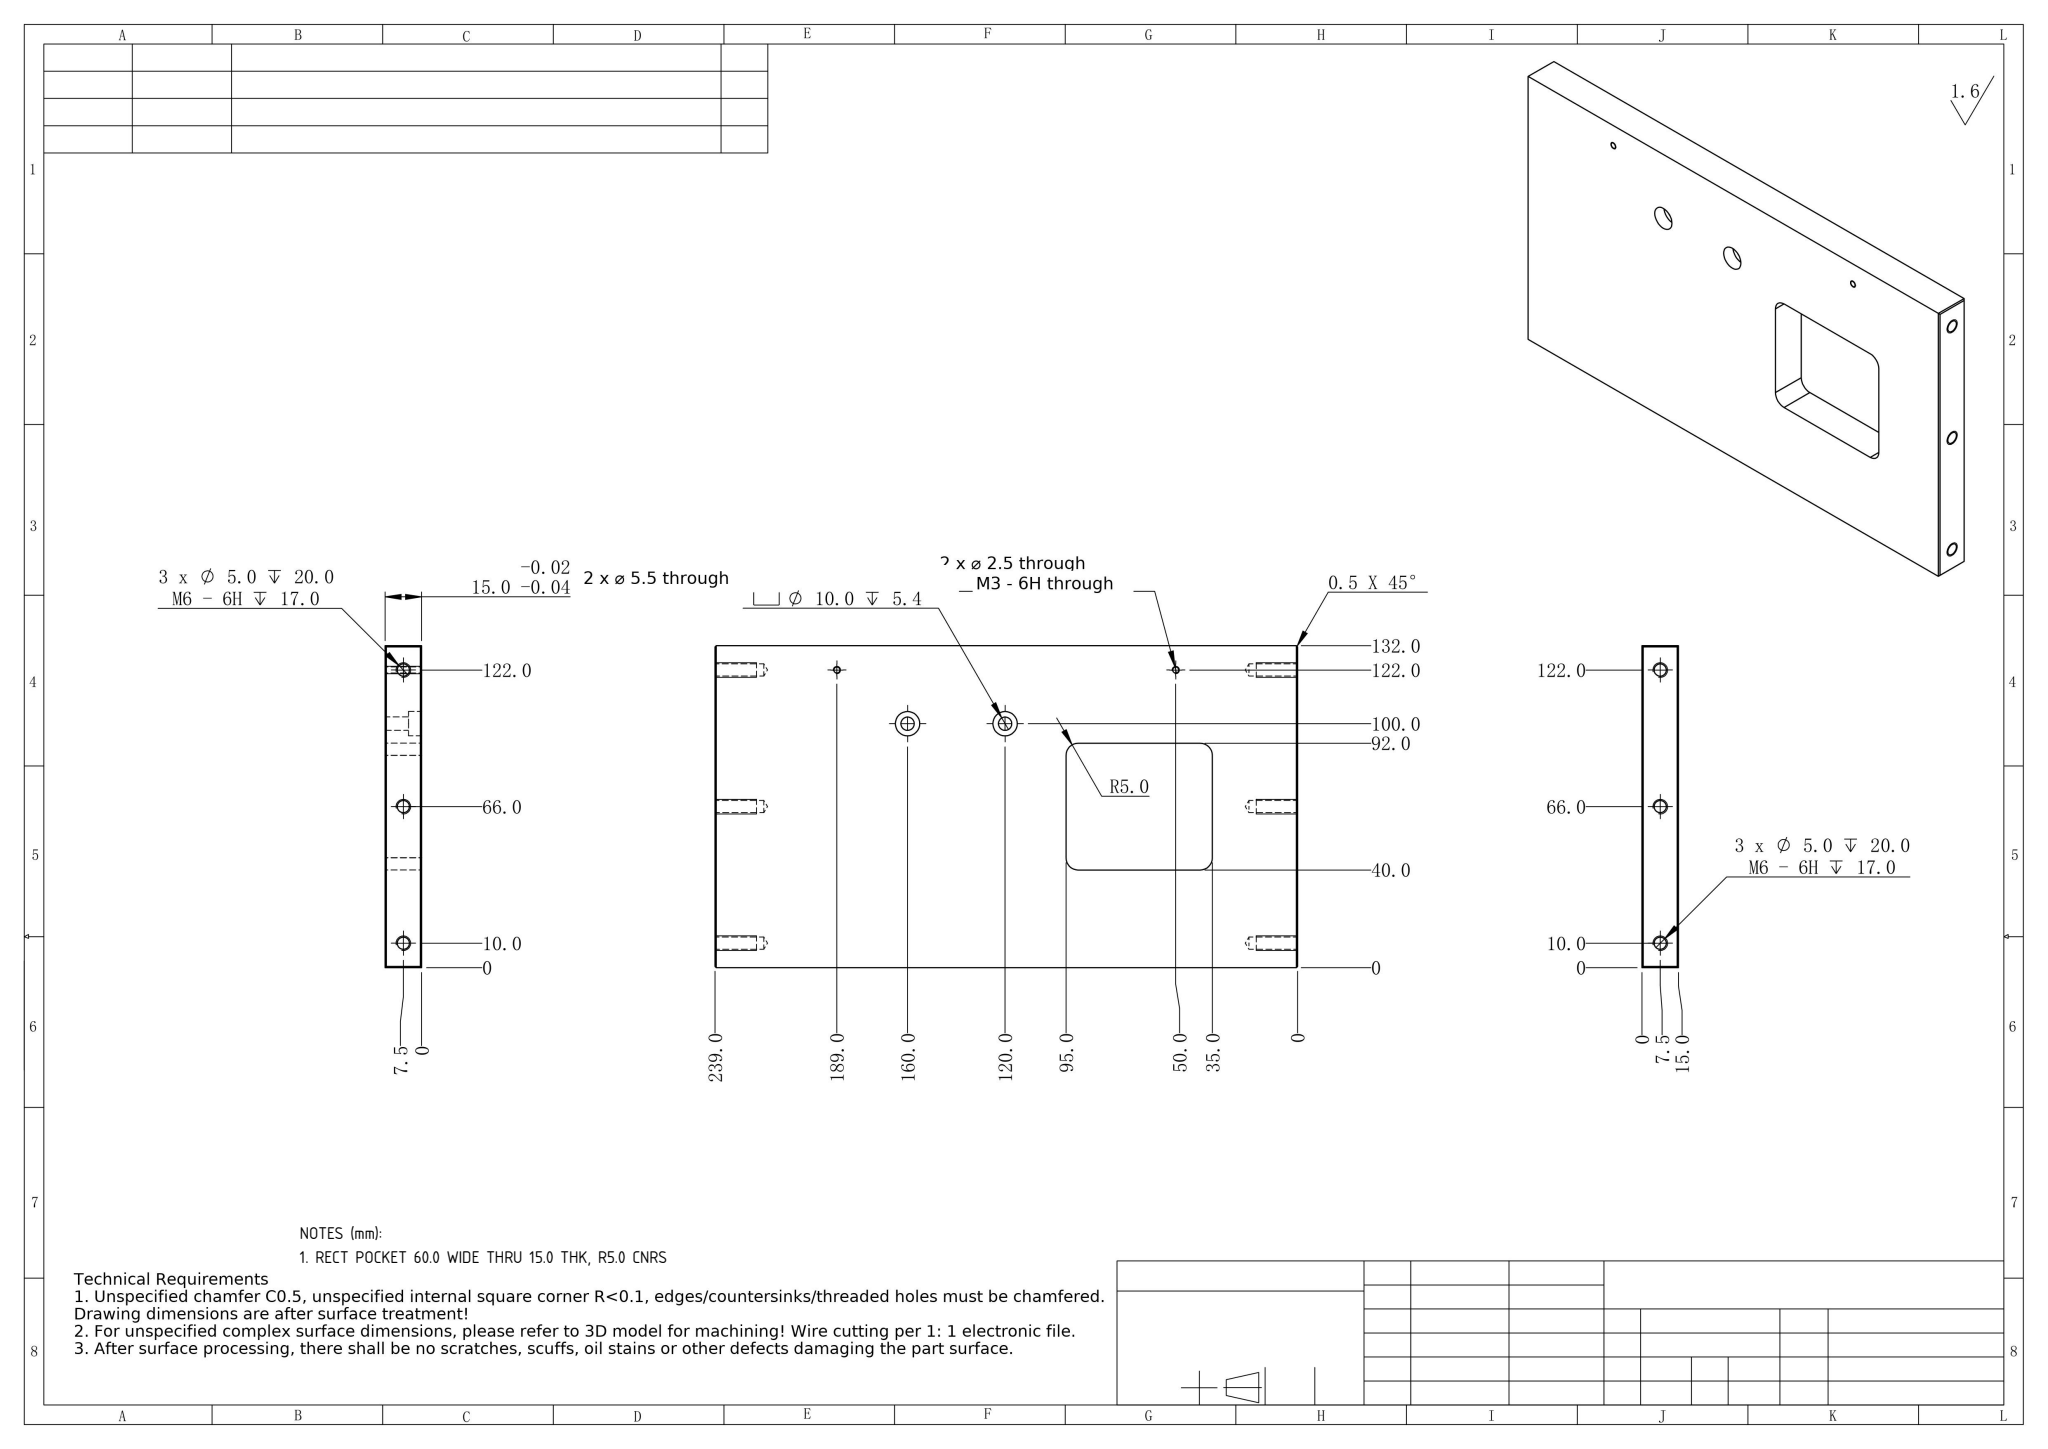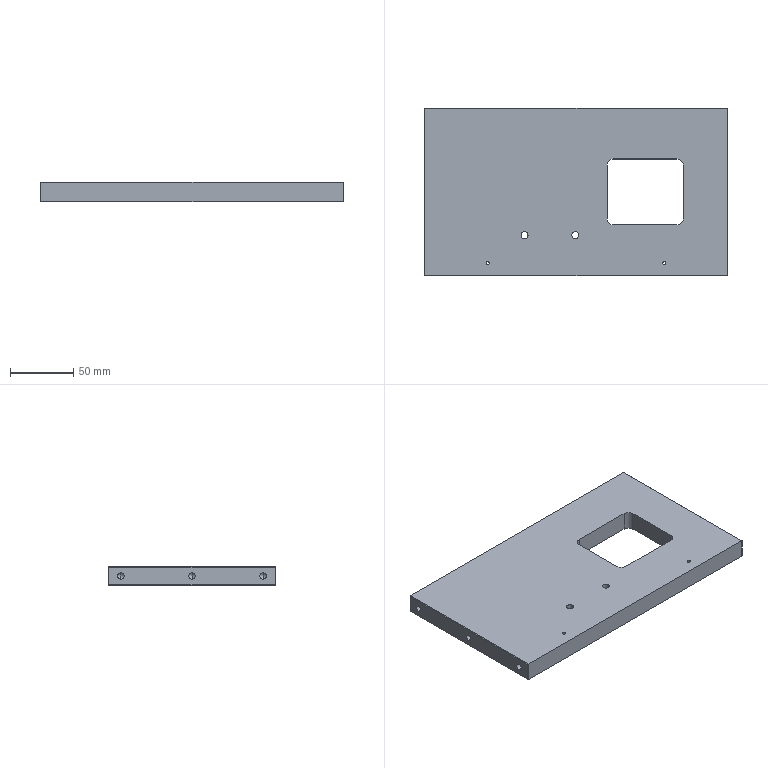Part | SolidWorks | mm | 1 solid | 60 faces | box 239 x 132 x 15 mm | volume 422802 mm3 | cylinder 28 | plane 20 | cone 12 | commonest cylinder face diameters 5 x12 10 x8 2.5 x4 5.5 x4
Drawing notes:
RECT POCKET 60.0 WIDE THRU 15.0 THK, R5.0 CNRS | from the solid: x-planes 144.0/204.0 (95.0 & 35.0 from x=239 datum) give 60.0 width; corner cyls Ø10 at (149/199, 45/87) length 15.0 = full thk; y-planes 40.0/92.0; no intermediate z floor
build123d program:
from build123d import *

# Parameters (mm, degrees)
SKETCH1_W                                       = 239
SKETCH1_H                                       = 132
BOSS_EXTRUDE1_DEPTH                             = 7.5
M6_TAPPED_HOLE1_D                               = 5
M6_TAPPED_HOLE1_DEPTH                           = 20
M6_TAPPED_HOLE1_TIP                             = 1.502
M6_TAPPED_HOLE2_D                               = 5
M6_TAPPED_HOLE2_DEPTH                           = 20
M6_TAPPED_HOLE2_TIP                             = 1.502
M5_HEX_SOCKET_HEAD_CAP_SCREW_CBORE1_D           = 5.5
M5_HEX_SOCKET_HEAD_CAP_SCREW_CBORE1_CBORE_D     = 10
M5_HEX_SOCKET_HEAD_CAP_SCREW_CBORE1_CBORE_DEPTH = 5.4
M3_TAPPED_HOLE1_D                               = 2.5
SKETCH10_W                                      = 60
SKETCH10_H                                      = 52
CUT_EXTRUDE1_DEPTH                              = 274.441
FILLET1_R                                       = 5
CHAMFER1_SIZE                                   = 0.5


with BuildPart() as part:
    # Sketch1 → Boss-Extrude1 (new, symmetric)
    with BuildSketch(Plane.XY):
        with Locations((119.5, 66)):
            Rectangle(SKETCH1_W, SKETCH1_H)
    extrude(amount=BOSS_EXTRUDE1_DEPTH, both=True)

    # M6 Tapped Hole1
    with Locations(Plane(origin=(239, 0, 0), x_dir=(0, 0, -1), z_dir=(1, 0, 0))):
        with Locations((0, 122), (0, 66), (0, 10)):
            Hole(M6_TAPPED_HOLE1_D / 2, depth=M6_TAPPED_HOLE1_DEPTH)
            with Locations((0, 0, -(M6_TAPPED_HOLE1_DEPTH + M6_TAPPED_HOLE1_TIP / 2))):  # 118° drill point
                Cone(0, M6_TAPPED_HOLE1_D / 2, M6_TAPPED_HOLE1_TIP, mode=Mode.SUBTRACT)

    # M6 Tapped Hole2
    with Locations(Plane.ZY):
        with Locations((0, 122), (0, 66), (0, 10)):
            Hole(M6_TAPPED_HOLE2_D / 2, depth=M6_TAPPED_HOLE2_DEPTH)
            with Locations((0, 0, -(M6_TAPPED_HOLE2_DEPTH + M6_TAPPED_HOLE2_TIP / 2))):  # 118° drill point
                Cone(0, M6_TAPPED_HOLE2_D / 2, M6_TAPPED_HOLE2_TIP, mode=Mode.SUBTRACT)

    # M5 Hex Socket Head Cap Screw CBORE1 (through all)
    with Locations(Plane(origin=(0, 0, -7.5), x_dir=(-1, 0, 0), z_dir=(0, 0, -1))):
        with Locations((-79, 32), (-119, 32)):
            CounterBoreHole(M5_HEX_SOCKET_HEAD_CAP_SCREW_CBORE1_D / 2, M5_HEX_SOCKET_HEAD_CAP_SCREW_CBORE1_CBORE_D / 2, M5_HEX_SOCKET_HEAD_CAP_SCREW_CBORE1_CBORE_DEPTH)

    # M3 Tapped Hole1 (through all)
    with Locations(Plane(origin=(0, 0, -7.5), x_dir=(-1, 0, 0), z_dir=(0, 0, -1))):
        with Locations((-50, 10), (-189, 10)):
            Hole(M3_TAPPED_HOLE1_D / 2)

    # Sketch10 → Cut-Extrude1 (cut, through all)
    with BuildSketch(Plane.XY.offset(7.5)):
        with Locations((174, 66)):
            Rectangle(SKETCH10_W, SKETCH10_H)
    extrude(amount=-CUT_EXTRUDE1_DEPTH, mode=Mode.SUBTRACT)

    # Fillet1
    fillet1_edges = [part.edges().sort_by_distance(p)[0] for p in [
        (144, 40, 0),
        (144, 92, 0),
        (204, 92, 0),
        (204, 40, 0),
    ]]
    fillet(fillet1_edges, radius=FILLET1_R)

    # Chamfer1
    chamfer1_edges = [part.edges().sort_by_distance(p)[0] for p in [
        (239, 66, 7.5),
        (0, 66, 7.5),
        (239, 66, -7.5),
        (0, 66, -7.5),
        (0, 132, 0),
        (239, 132, 0),
        (239, 0, 0),
        (0, 0, 0),
    ]]
    chamfer(chamfer1_edges, length=CHAMFER1_SIZE)


solid = part.part